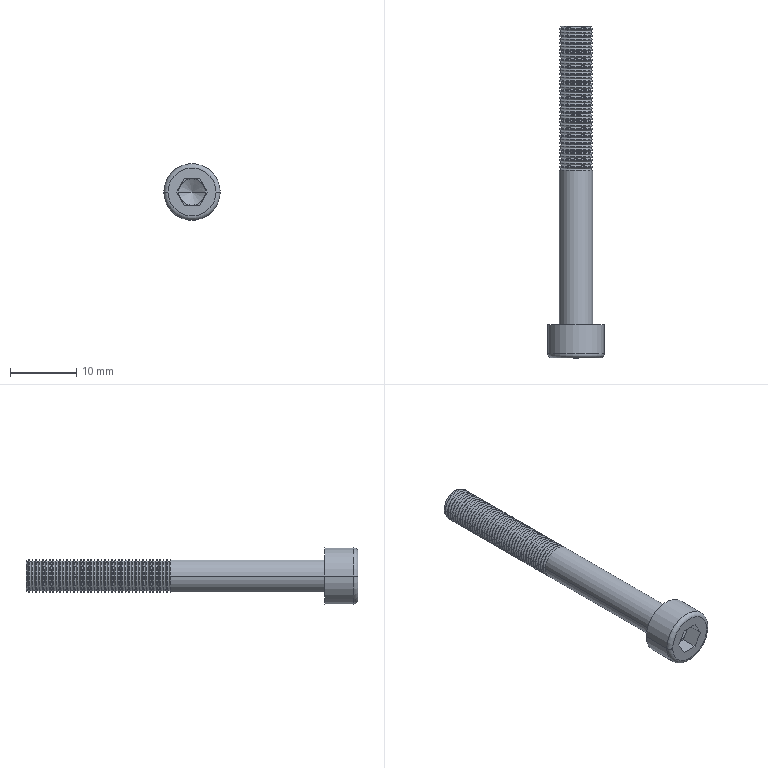Component | SolidWorks | LongSideClampingAssemblyBGeneralAssembly-1_HexSocketHeadCap-M5X45-0510-3 | 1 solid | 275 faces | box 8.5 x 50 x 8.5 mm | volume 1075 mm3 | cone 172 | cylinder 86 | plane 15 | torus 2 | commonest cylinder face diameters 5 x84 8.5 x2
build123d program:
from build123d import *

# Parameters (mm, degrees)
SKETCH1_R           = 4.25
BASEHEAD_DEPTH      = 5
SKETCH2_R           = 2.5
BASEBODY_DEPTH      = 45
HEXAGONSOCKET_DEPTH = 2.5
TOPFILLET_R         = 0.625
CHAMFER1_SIZE       = 0.2
LPATTERN10_COUNT    = 42
LPATTERN10_PITCH    = 0.5196


with BuildPart() as part:
    # Sketch1 → BaseHead (new body)
    with BuildSketch(Plane(origin=(0, 0, 0), x_dir=(0, 0, -1), z_dir=(1, 0, 0))):
        Circle(SKETCH1_R)
    extrude(amount=BASEHEAD_DEPTH)

    # Sketch2 → BaseBody (add)
    with BuildSketch(Plane(origin=(5, 0, 0), x_dir=(0, 0, -1), z_dir=(1, 0, 0))):
        with Locations(Location((0, 0, 0), (0, 0, 180))):
            Circle(SKETCH2_R)
    extrude(amount=BASEBODY_DEPTH)

    # Sketch3 → HexagonSocket (cut)
    with BuildSketch(Plane(origin=(0, 0, 0), x_dir=(0, 0, -1), z_dir=(1, 0, 0))):
        Polygon((2.309, 0), (1.155, 2), (-1.155, 2), (-2.309, 0), (-1.155, -2), (1.155, -2), align=None)
    extrude(amount=HEXAGONSOCKET_DEPTH, mode=Mode.SUBTRACT)

    # Sketch4 → Cut-Revolve1 (revolve, cut)
    with BuildSketch(Plane(origin=(-4.196, 0.75, 0), x_dir=(-1, 0, 0), z_dir=(0, 0, 1)), mode=Mode.PRIVATE) as cut_revolve1_sk:
        Polygon((-6.696, 2.75), (-7.851, 0.75), (-6.696, 0.75), align=None)
    revolve(cut_revolve1_sk.sketch.rotate(Axis((0.839, 0, 0), (-1, 0, 0)), 90), axis=Axis((0.839, 0, 0), (-1, 0, 0)), mode=Mode.SUBTRACT)

    # TopFillet
    topfillet_edges = [part.edges().sort_by_distance(p)[0] for p in [
        (0, 0, 4.25),
    ]]
    fillet(topfillet_edges, radius=TOPFILLET_R)

    # Chamfer1
    chamfer1_edges = [part.edges().sort_by_distance(p)[0] for p in [
        (50, 0, -2.5),
    ]]
    chamfer(chamfer1_edges, length=CHAMFER1_SIZE)

    # Sketch5 → Cut-Revolve10 (revolve, cut)
    with BuildSketch(Plane.XY, mode=Mode.PRIVATE) as cut_revolve10_sk:
        Polygon((49.8, 2.125), (50.017, 2.5), (50.017, 2.933), (49.584, 2.933), (49.584, 2.5), align=None)
    cut_revolve10 = revolve(cut_revolve10_sk.sketch.rotate(Axis((0, 0, 0), (1, 0, 0)), 90), axis=Axis((0, 0, 0), (1, 0, 0)), mode=Mode.SUBTRACT)

    # LPattern10: Cut-Revolve10 ×42
    with Locations(*[(-i * LPATTERN10_PITCH, 0, 0) for i in range(1, LPATTERN10_COUNT)]):
        add(cut_revolve10, mode=Mode.SUBTRACT)


solid = part.part

# Placed as in the assembly
solid = solid.moved(Location((-3150.658, -141.909, 3570), (90, 90, 0)))